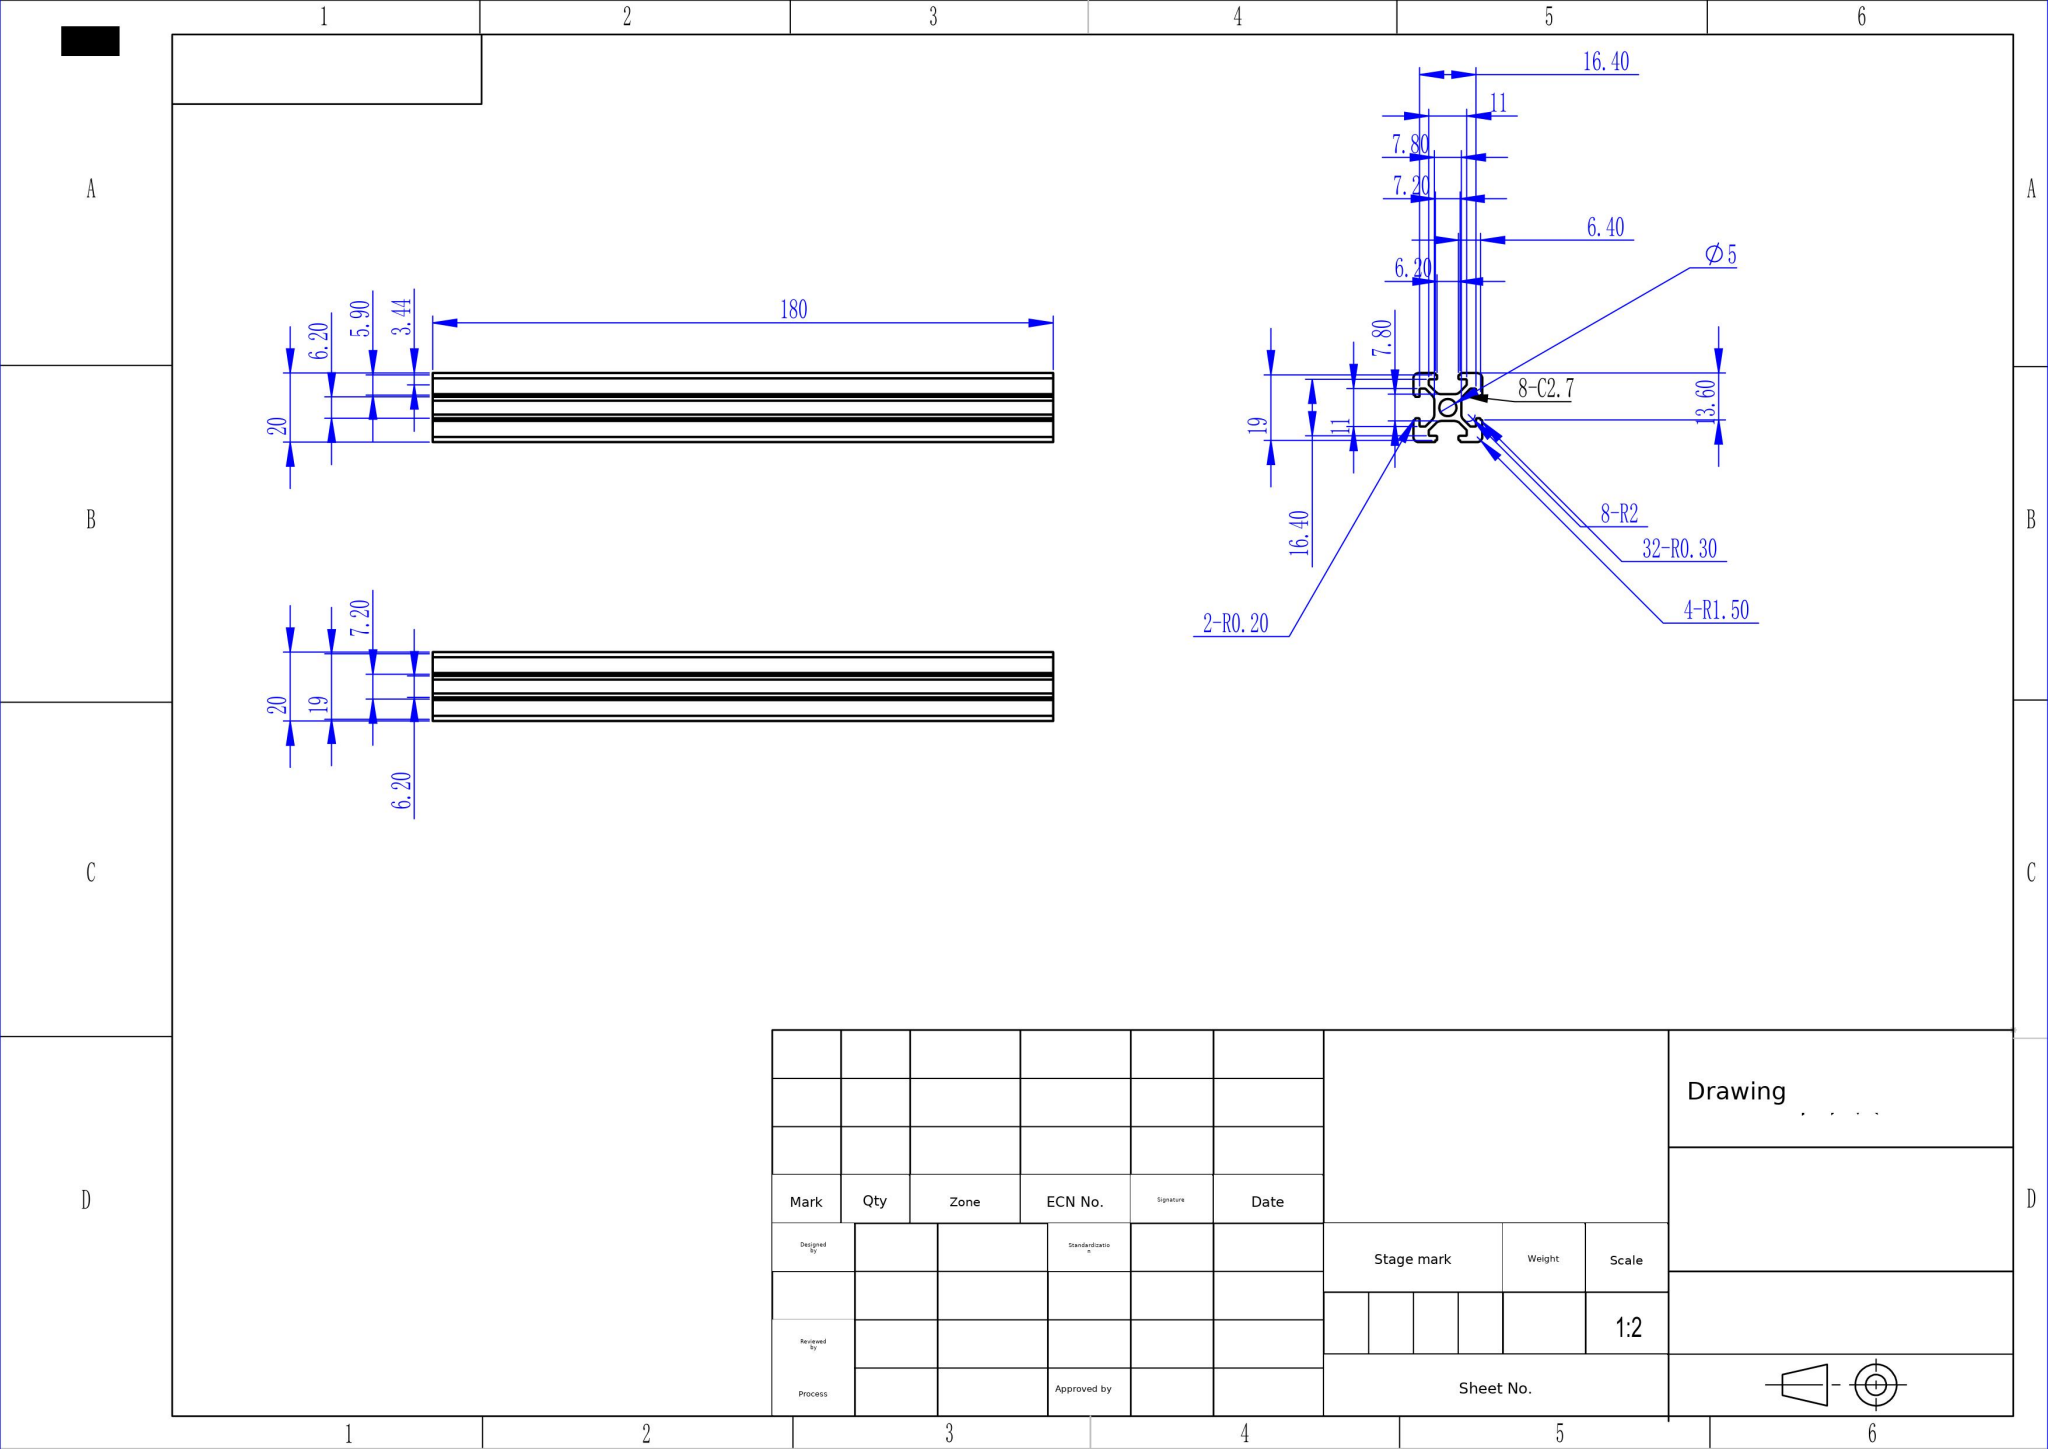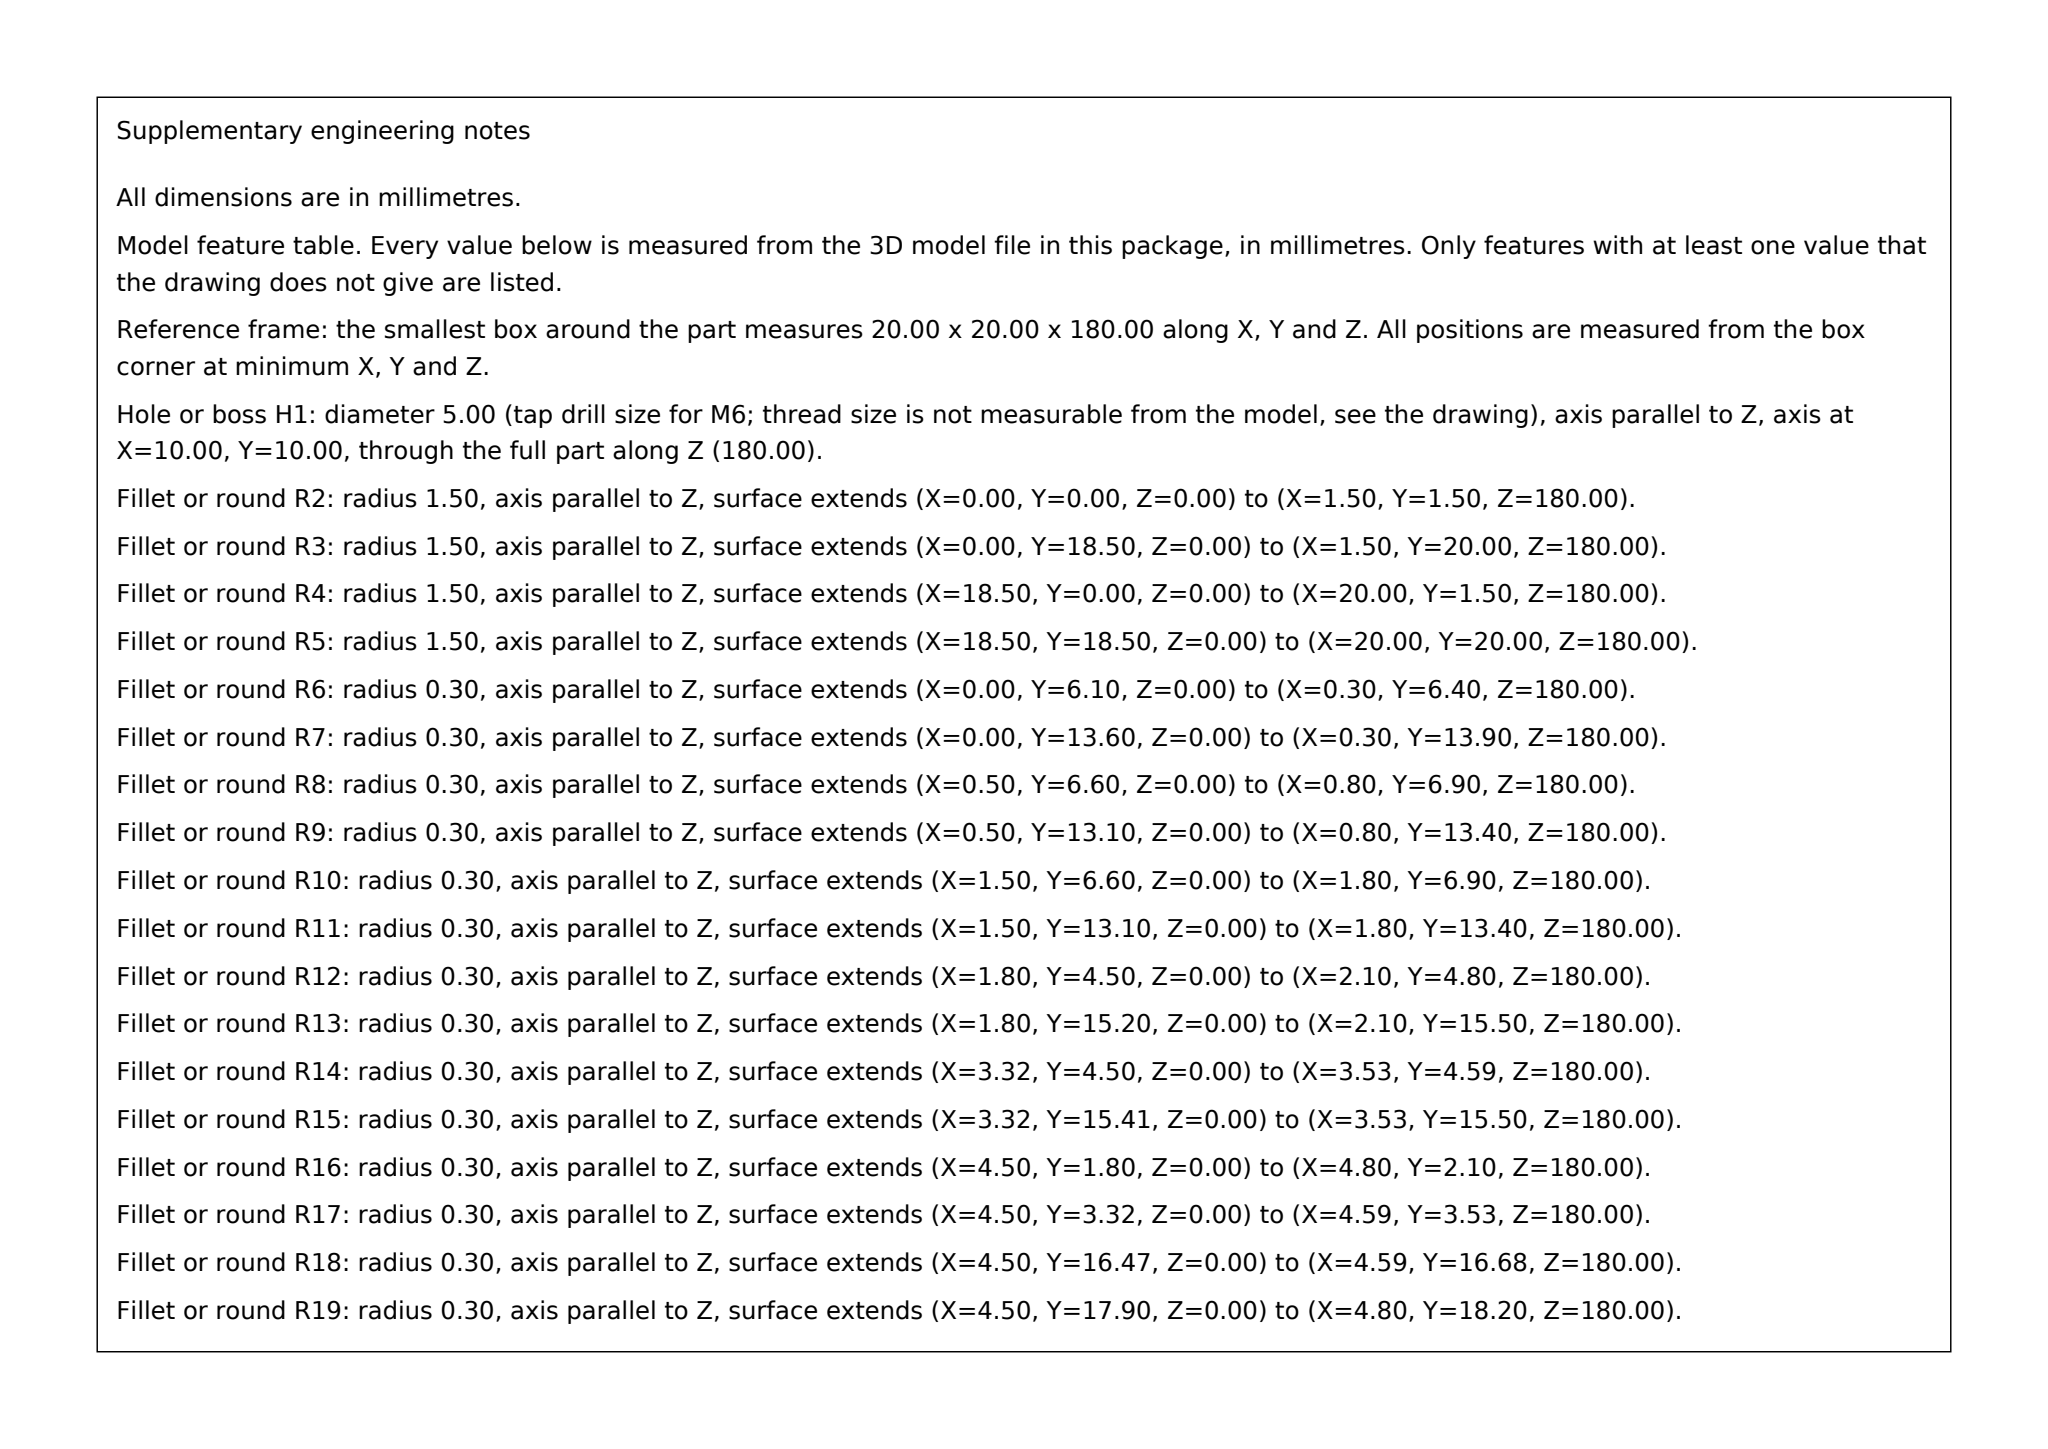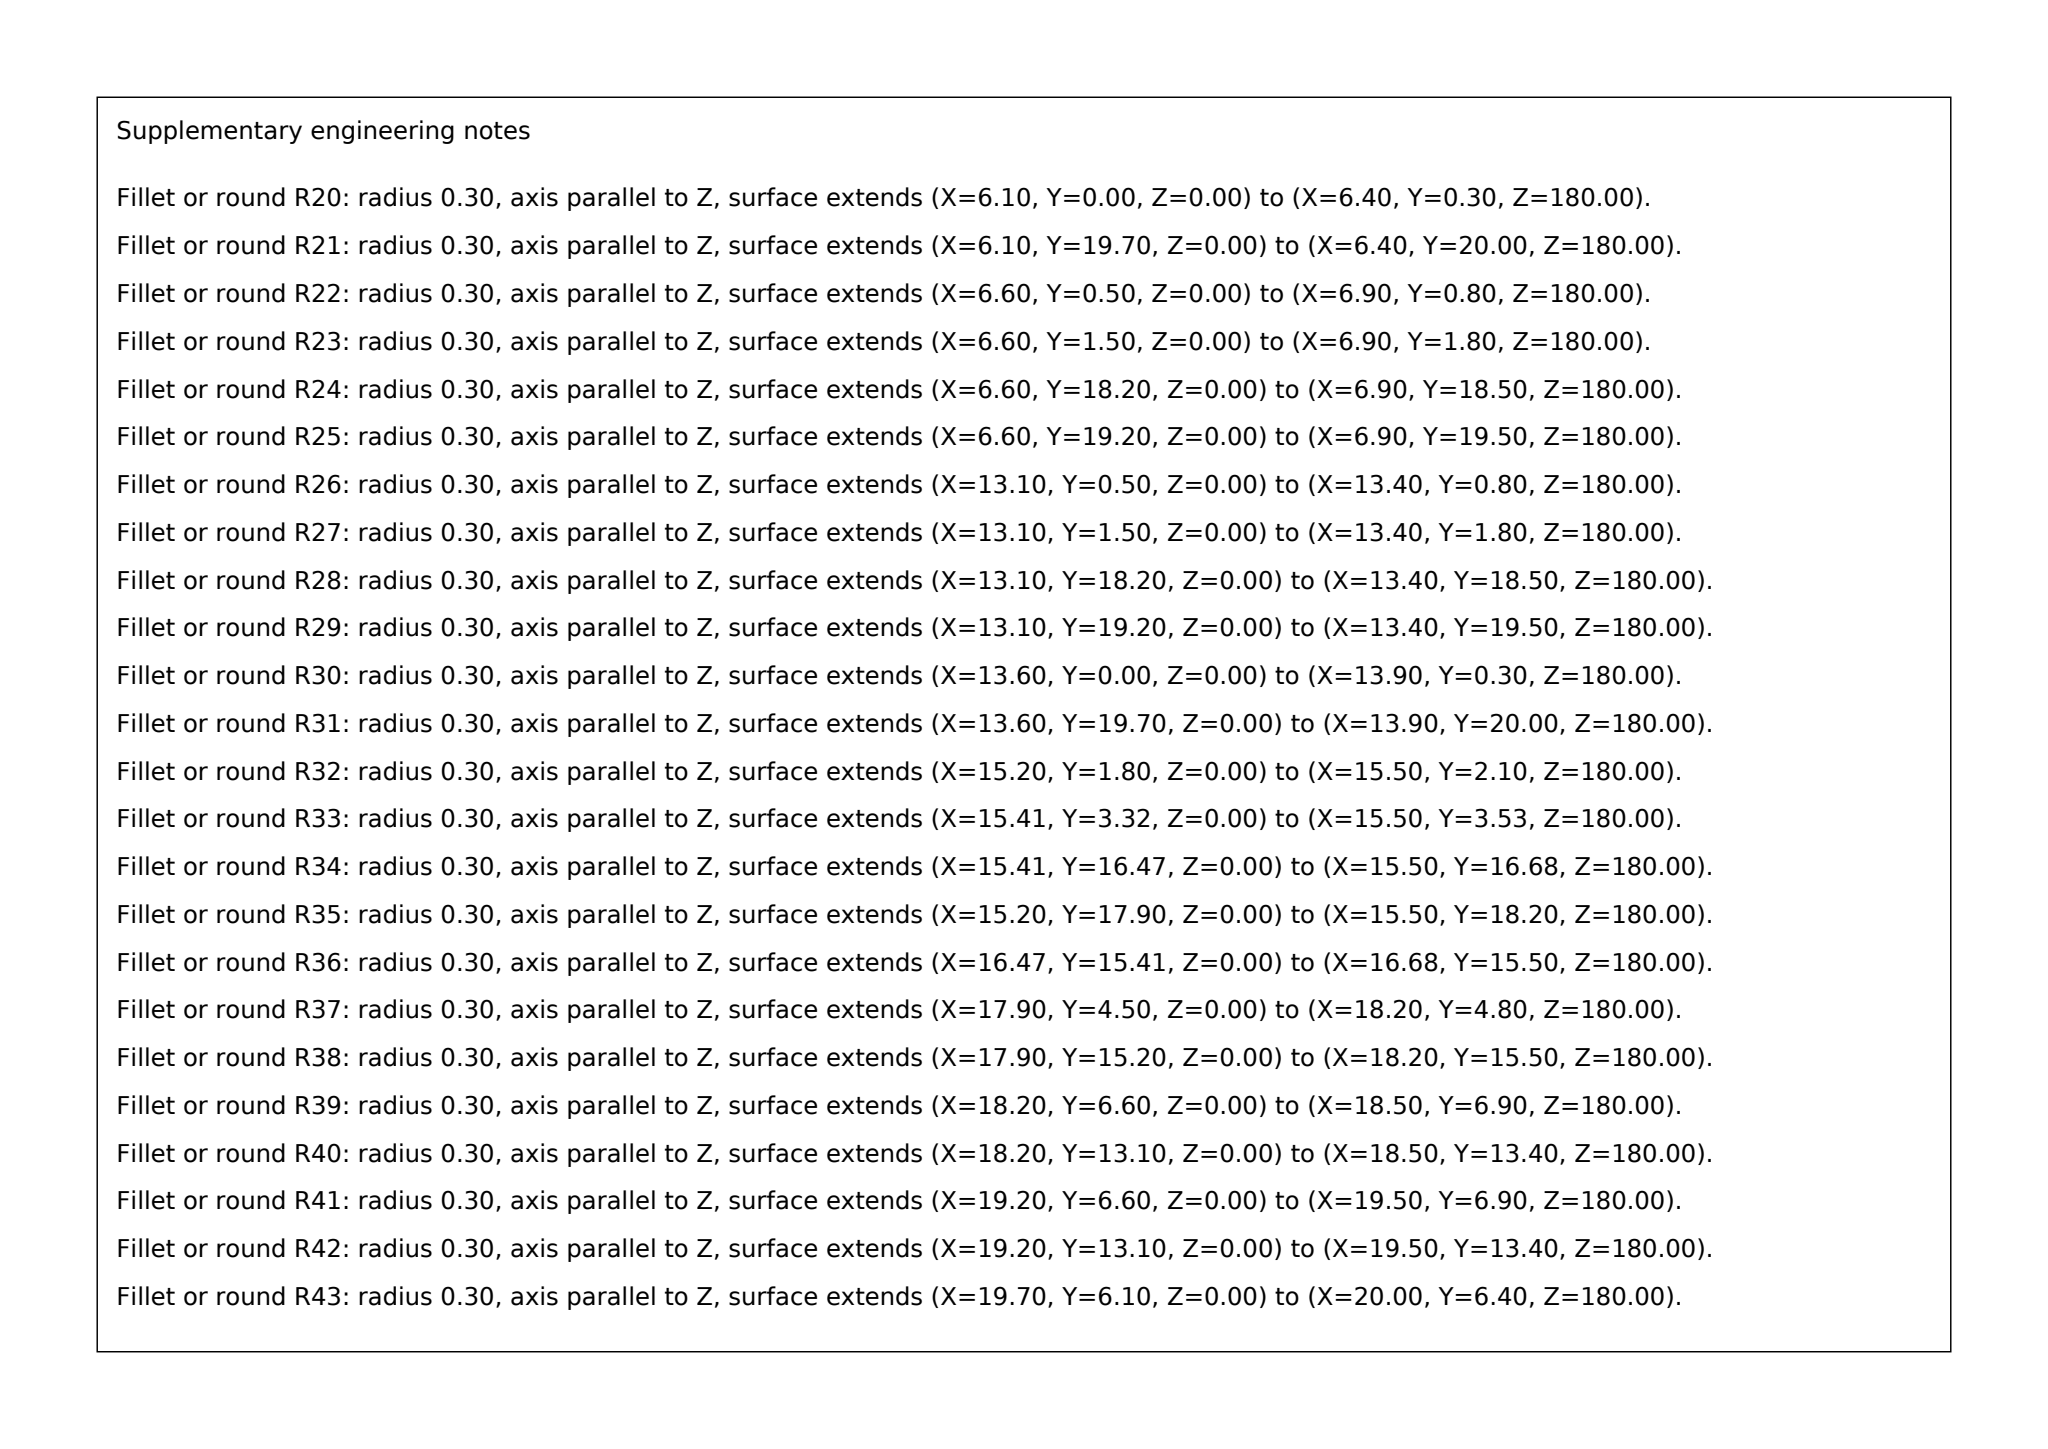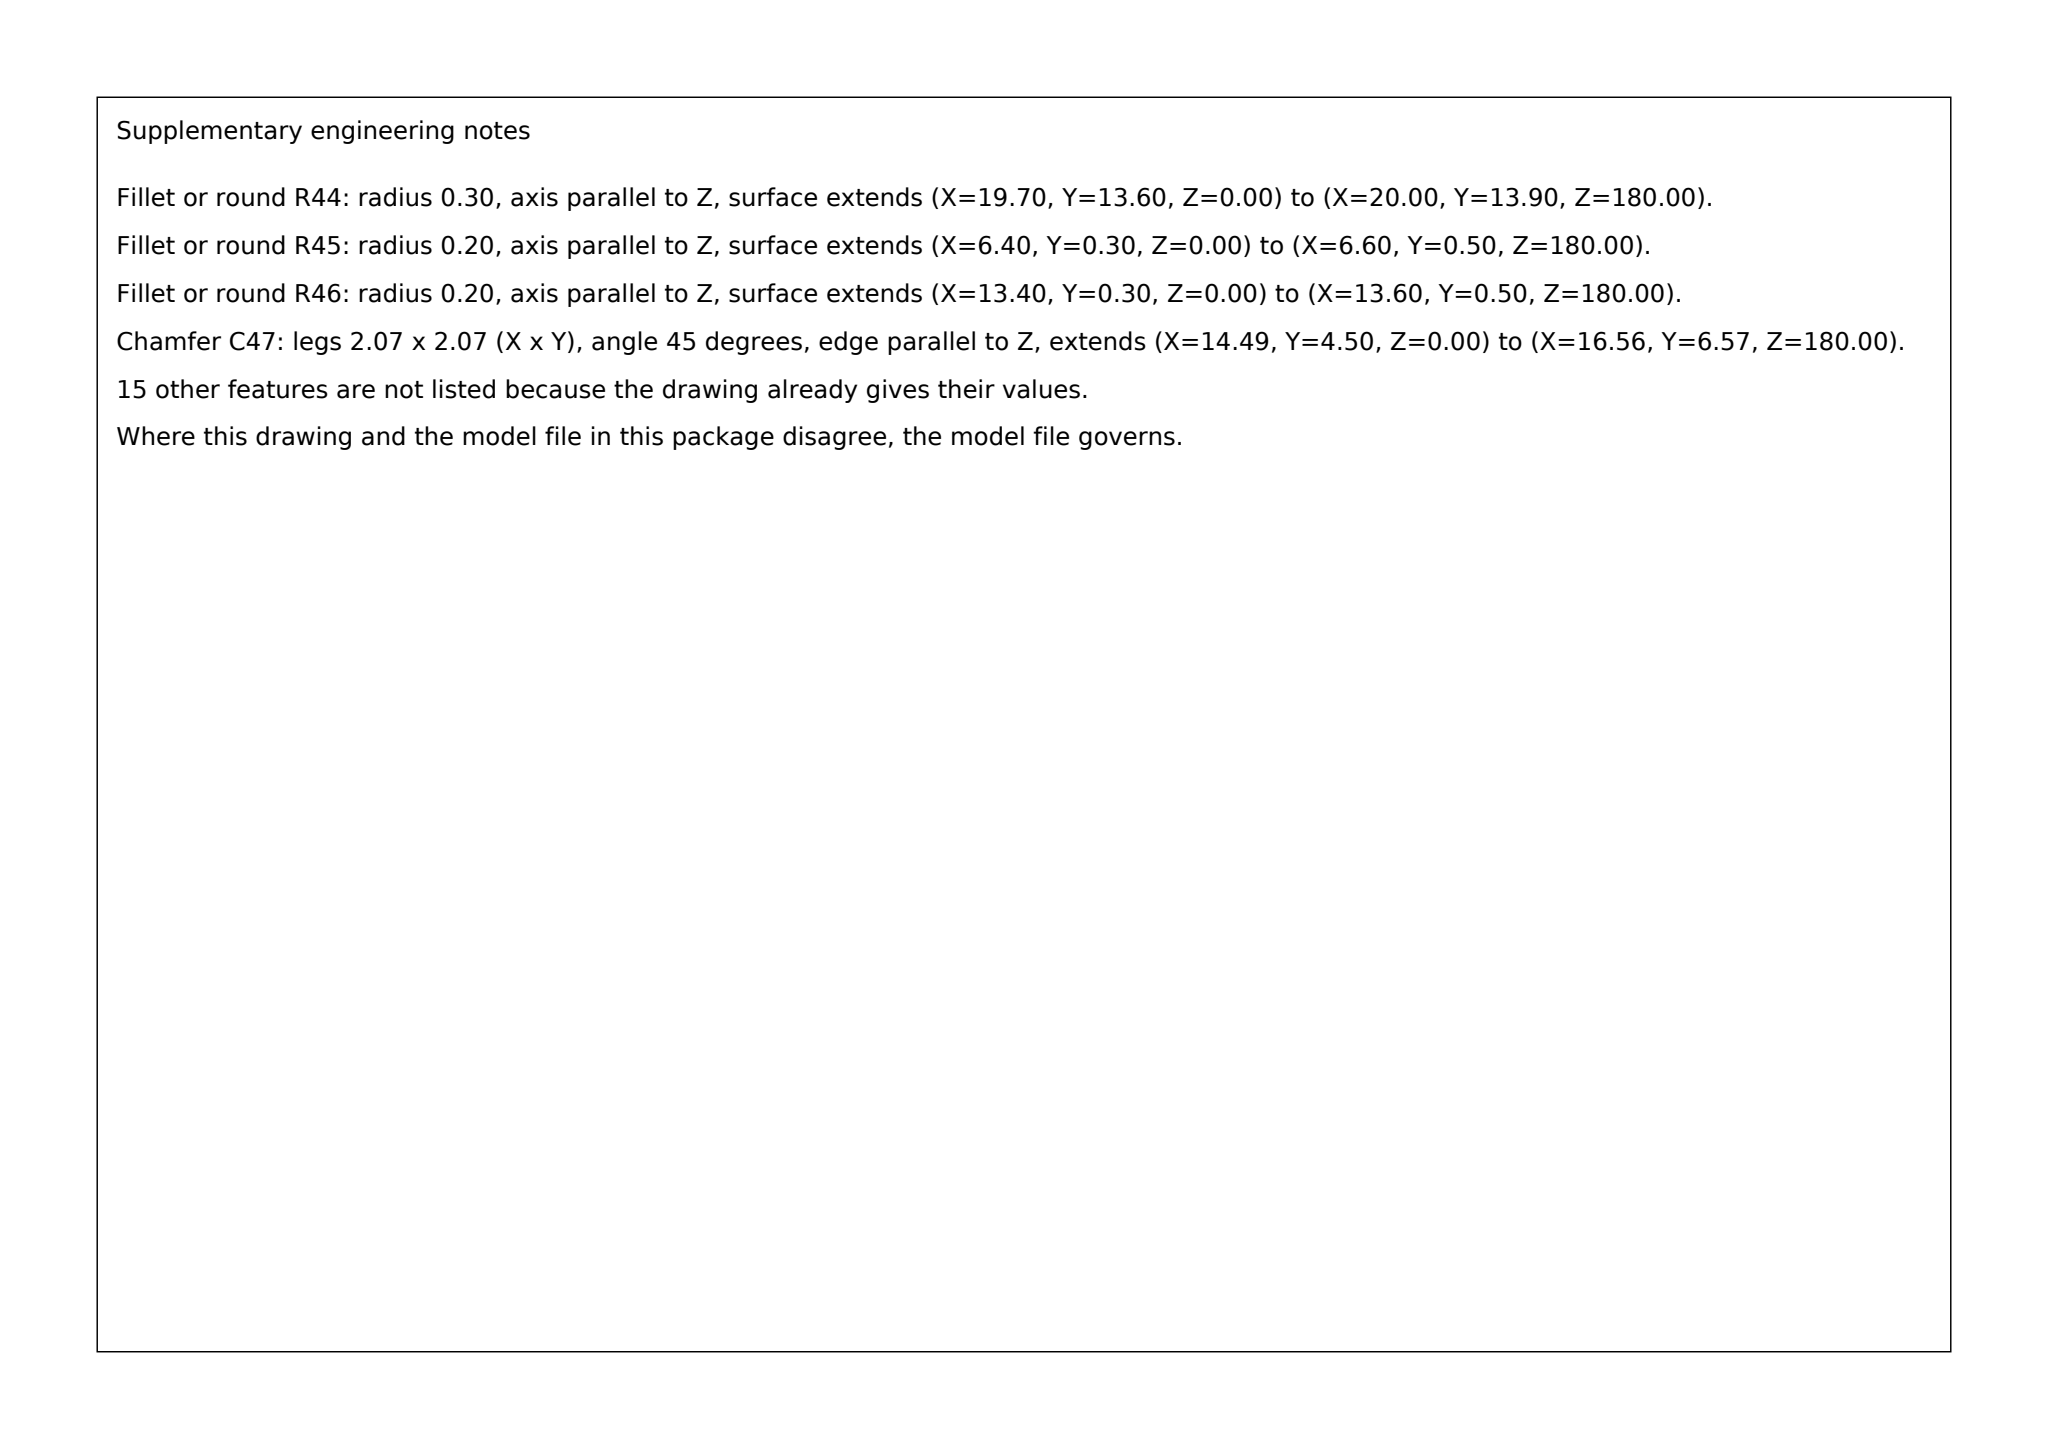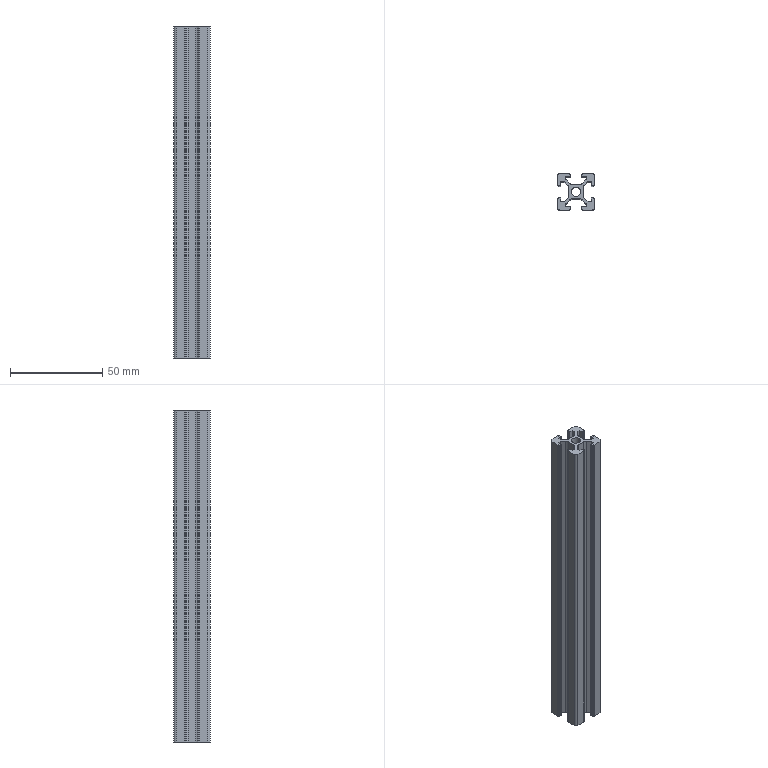Part | SolidWorks | mm | 1 solid | 113 faces | box 20 x 20 x 180 mm | volume 30838 mm3 | plane 58 | cylinder 55 | commonest cylinder face diameters 0.6 x39 4 x8 3 x4 5 x2 0.4 x2
build123d program:
from build123d import *

# Parameters (mm, degrees)
SKETCH1_R           = 2.5
BOSS_EXTRUDE1_DEPTH = 180


with BuildPart() as part:
    # Sketch1 → Boss-Extrude1 (new body)
    with BuildSketch(Plane(origin=(0, 0, 0), x_dir=(-1, 0, 0), z_dir=(0, 0, -1))):
        with BuildLine():
            Line((-5845.236, 2818.35), (-5845.236, 2820.15))
            ThreePointArc((-5845.236, 2820.15), (-5845.323, 2820.362), (-5845.536, 2820.45))
            Line((-5845.536, 2820.45), (-5846.236, 2820.45))
            ThreePointArc((-5846.236, 2820.45), (-5846.448, 2820.362), (-5846.536, 2820.15))
            Line((-5846.536, 2820.15), (-5846.536, 2819.95))
            Line((-5846.536, 2819.95), (-5846.736, 2819.95))
            ThreePointArc((-5846.736, 2819.95), (-5846.948, 2819.862), (-5847.036, 2819.65))
            Line((-5847.036, 2819.65), (-5847.036, 2815.05))
            ThreePointArc((-5847.036, 2815.05), (-5846.596, 2813.989), (-5845.536, 2813.55))
            Line((-5845.536, 2813.55), (-5840.936, 2813.55))
            ThreePointArc((-5840.936, 2813.55), (-5840.723, 2813.638), (-5840.636, 2813.85))
            ThreePointArc((-5840.636, 2813.85), (-5840.577, 2813.991), (-5840.436, 2814.05))
            ThreePointArc((-5840.436, 2814.05), (-5840.223, 2814.138), (-5840.136, 2814.35))
            Line((-5840.136, 2814.35), (-5840.136, 2815.05))
            ThreePointArc((-5840.136, 2815.05), (-5840.223, 2815.262), (-5840.436, 2815.35))
            Line((-5840.436, 2815.35), (-5842.236, 2815.35))
            ThreePointArc((-5842.236, 2815.35), (-5842.448, 2815.438), (-5842.536, 2815.65))
            Line((-5842.536, 2815.65), (-5842.536, 2816.865))
            ThreePointArc((-5842.536, 2816.865), (-5842.513, 2816.98), (-5842.448, 2817.077))
            Line((-5842.448, 2817.077), (-5840.461, 2819.064))
            ThreePointArc((-5840.461, 2819.064), (-5839.812, 2819.498), (-5839.046, 2819.65))
            Line((-5839.046, 2819.65), (-5835.025, 2819.65))
            ThreePointArc((-5835.025, 2819.65), (-5834.259, 2819.498), (-5833.61, 2819.064))
            Line((-5833.61, 2819.064), (-5831.623, 2817.077))
            ThreePointArc((-5831.623, 2817.077), (-5831.558, 2816.98), (-5831.536, 2816.865))
            Line((-5831.536, 2816.865), (-5831.536, 2815.65))
            ThreePointArc((-5831.536, 2815.65), (-5831.623, 2815.438), (-5831.836, 2815.35))
            Line((-5831.836, 2815.35), (-5833.636, 2815.35))
            ThreePointArc((-5833.636, 2815.35), (-5833.848, 2815.262), (-5833.936, 2815.05))
            Line((-5833.936, 2815.05), (-5833.936, 2814.35))
            ThreePointArc((-5833.936, 2814.35), (-5833.848, 2814.138), (-5833.636, 2814.05))
            ThreePointArc((-5833.636, 2814.05), (-5833.494, 2813.991), (-5833.436, 2813.85))
            ThreePointArc((-5833.436, 2813.85), (-5833.348, 2813.638), (-5833.136, 2813.55))
            Line((-5833.136, 2813.55), (-5828.536, 2813.55))
            ThreePointArc((-5828.536, 2813.55), (-5827.475, 2813.989), (-5827.036, 2815.05))
            Line((-5827.036, 2815.05), (-5827.036, 2819.65))
            ThreePointArc((-5827.036, 2819.65), (-5827.123, 2819.862), (-5827.336, 2819.95))
            Line((-5827.336, 2819.95), (-5827.536, 2819.95))
            Line((-5827.536, 2819.95), (-5827.536, 2820.15))
            ThreePointArc((-5827.536, 2820.15), (-5827.623, 2820.362), (-5827.836, 2820.45))
            Line((-5827.836, 2820.45), (-5828.536, 2820.45))
            ThreePointArc((-5828.536, 2820.45), (-5828.748, 2820.362), (-5828.836, 2820.15))
            Line((-5828.836, 2820.15), (-5828.836, 2818.35))
            ThreePointArc((-5828.836, 2818.35), (-5828.923, 2818.138), (-5829.136, 2818.05))
            Line((-5829.136, 2818.05), (-5830.351, 2818.05))
            ThreePointArc((-5830.351, 2818.05), (-5830.465, 2818.073), (-5830.563, 2818.138))
            Line((-5830.563, 2818.138), (-5832.55, 2820.125))
            ThreePointArc((-5832.55, 2820.125), (-5832.983, 2820.774), (-5833.136, 2821.539))
            Line((-5833.136, 2821.539), (-5833.136, 2825.561))
            ThreePointArc((-5833.136, 2825.561), (-5832.983, 2826.326), (-5832.55, 2826.975))
            Line((-5832.55, 2826.975), (-5830.563, 2828.962))
            ThreePointArc((-5830.563, 2828.962), (-5830.465, 2829.027), (-5830.351, 2829.05))
            Line((-5830.351, 2829.05), (-5829.136, 2829.05))
            ThreePointArc((-5829.136, 2829.05), (-5828.923, 2828.962), (-5828.836, 2828.75))
            Line((-5828.836, 2828.75), (-5828.836, 2826.95))
            ThreePointArc((-5828.836, 2826.95), (-5828.748, 2826.738), (-5828.536, 2826.65))
            Line((-5828.536, 2826.65), (-5827.836, 2826.65))
            ThreePointArc((-5827.836, 2826.65), (-5827.623, 2826.738), (-5827.536, 2826.95))
            Line((-5827.536, 2826.95), (-5827.536, 2827.15))
            Line((-5827.536, 2827.15), (-5827.336, 2827.15))
            ThreePointArc((-5827.336, 2827.15), (-5827.123, 2827.238), (-5827.036, 2827.45))
            Line((-5827.036, 2827.45), (-5827.036, 2832.05))
            ThreePointArc((-5827.036, 2832.05), (-5827.475, 2833.11), (-5828.536, 2833.55))
            Line((-5828.536, 2833.55), (-5833.136, 2833.55))
            ThreePointArc((-5833.136, 2833.55), (-5833.348, 2833.462), (-5833.436, 2833.25))
            Line((-5833.436, 2833.25), (-5833.436, 2833.05))
            Line((-5833.436, 2833.05), (-5833.636, 2833.05))
            ThreePointArc((-5833.636, 2833.05), (-5833.848, 2832.962), (-5833.936, 2832.75))
            Line((-5833.936, 2832.75), (-5833.936, 2832.05))
            ThreePointArc((-5833.936, 2832.05), (-5833.848, 2831.838), (-5833.636, 2831.75))
            Line((-5833.636, 2831.75), (-5831.836, 2831.75))
            ThreePointArc((-5831.836, 2831.75), (-5831.623, 2831.662), (-5831.536, 2831.45))
            Line((-5831.536, 2831.45), (-5831.536, 2830.235))
            ThreePointArc((-5831.536, 2830.235), (-5831.558, 2830.12), (-5831.623, 2830.023))
            Line((-5831.623, 2830.023), (-5833.61, 2828.036))
            ThreePointArc((-5833.61, 2828.036), (-5834.259, 2827.602), (-5835.025, 2827.45))
            Line((-5835.025, 2827.45), (-5839.046, 2827.45))
            ThreePointArc((-5839.046, 2827.45), (-5839.812, 2827.602), (-5840.461, 2828.036))
            Line((-5840.461, 2828.036), (-5842.448, 2830.023))
            ThreePointArc((-5842.448, 2830.023), (-5842.513, 2830.12), (-5842.536, 2830.235))
            Line((-5842.536, 2830.235), (-5842.536, 2831.45))
            ThreePointArc((-5842.536, 2831.45), (-5842.448, 2831.662), (-5842.236, 2831.75))
            Line((-5842.236, 2831.75), (-5840.436, 2831.75))
            ThreePointArc((-5840.436, 2831.75), (-5840.223, 2831.838), (-5840.136, 2832.05))
            Line((-5840.136, 2832.05), (-5840.136, 2832.75))
            ThreePointArc((-5840.136, 2832.75), (-5840.223, 2832.962), (-5840.436, 2833.05))
            Line((-5840.436, 2833.05), (-5840.636, 2833.05))
            Line((-5840.636, 2833.05), (-5840.636, 2833.25))
            ThreePointArc((-5840.636, 2833.25), (-5840.723, 2833.462), (-5840.936, 2833.55))
            Line((-5840.936, 2833.55), (-5845.536, 2833.55))
            ThreePointArc((-5845.536, 2833.55), (-5846.596, 2833.11), (-5847.036, 2832.05))
            Line((-5847.036, 2832.05), (-5847.036, 2827.45))
            ThreePointArc((-5847.036, 2827.45), (-5846.948, 2827.238), (-5846.736, 2827.15))
            Line((-5846.736, 2827.15), (-5846.536, 2827.15))
            Line((-5846.536, 2827.15), (-5846.536, 2826.95))
            ThreePointArc((-5846.536, 2826.95), (-5846.448, 2826.738), (-5846.236, 2826.65))
            Line((-5846.236, 2826.65), (-5845.536, 2826.65))
            ThreePointArc((-5845.536, 2826.65), (-5845.323, 2826.738), (-5845.236, 2826.95))
            Line((-5845.236, 2826.95), (-5845.236, 2828.75))
            ThreePointArc((-5845.236, 2828.75), (-5845.148, 2828.962), (-5844.936, 2829.05))
            Line((-5844.936, 2829.05), (-5843.72, 2829.05))
            ThreePointArc((-5843.72, 2829.05), (-5843.606, 2829.027), (-5843.508, 2828.962))
            Line((-5843.508, 2828.962), (-5841.521, 2826.975))
            ThreePointArc((-5841.521, 2826.975), (-5841.088, 2826.326), (-5840.936, 2825.561))
            Line((-5840.936, 2825.561), (-5840.936, 2821.539))
            ThreePointArc((-5840.936, 2821.539), (-5841.088, 2820.774), (-5841.521, 2820.125))
            Line((-5841.521, 2820.125), (-5843.596, 2818.05))
            Line((-5843.596, 2818.05), (-5844.936, 2818.05))
            ThreePointArc((-5844.936, 2818.05), (-5845.148, 2818.138), (-5845.236, 2818.35))
        make_face()
        with Locations((-5837.036, 2823.55)):
            Circle(SKETCH1_R, mode=Mode.SUBTRACT)
    extrude(amount=-BOSS_EXTRUDE1_DEPTH)


solid = part.part